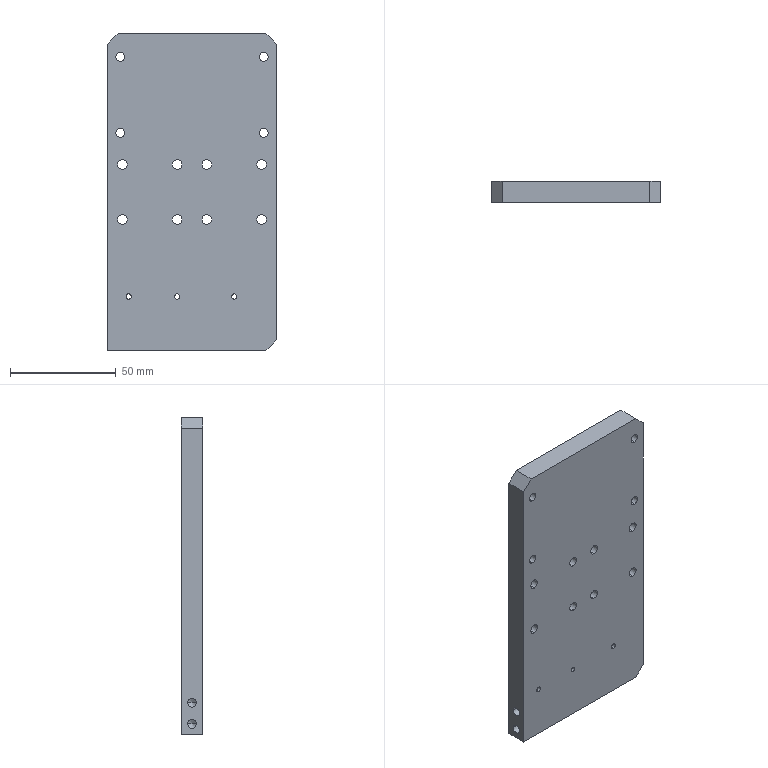Component | SolidWorks | F-YBExport-1-1_LSDH-6-025-1 | 1 solid | 79 faces | box 80 x 10 x 150 mm | volume 115928 mm3 | cylinder 54 | plane 17 | cone 8 | commonest cylinder face diameters 8 x16 4.5 x16 4.2 x12 2.5 x6 3 x4
build123d program:
from build123d import *

# Parameters (mm, degrees)
SKETCH1_W                                            = 150
SKETCH1_H                                            = 80
BOSS_EXTRUDE1_DEPTH                                  = 10
M3_TAPPED_HOLE1_D                                    = 2.5
HOLE_SIZE_ACCORDING_TO_THE_TYPE_OF_HEX_S_D           = 4.5
HOLE_SIZE_ACCORDING_TO_THE_TYPE_OF_HEX_S_CBORE_D     = 8
HOLE_SIZE_ACCORDING_TO_THE_TYPE_OF_HEX_S_CBORE_DEPTH = 4.6
M5_TAPPED_HOLE1_D                                    = 4.2
M5_TAPPED_HOLE1_DEPTH                                = 12.4
M5_TAPPED_HOLE1_TIP                                  = 1.262
M5_TAPPED_HOLE2_D                                    = 4.2
M5_TAPPED_HOLE2_DEPTH                                = 12.4
M5_TAPPED_HOLE2_TIP                                  = 1.262
F_3_0_3_DIAMETER_HOLE1_D                             = 3
F_3_0_3_DIAMETER_HOLE1_DEPTH                         = 7
F_3_0_3_DIAMETER_HOLE1_TIP                           = 0.9013
CHAMFER1_SIZE                                        = 5


with BuildPart() as part:
    # Sketch1 → Boss-Extrude1 (new body)
    with BuildSketch(Plane.XY):
        Rectangle(SKETCH1_W, SKETCH1_H)
    extrude(amount=BOSS_EXTRUDE1_DEPTH)

    # M3 Tapped Hole1 (through all)
    with Locations(Plane(origin=(49.5, 7, 10), x_dir=(1, 0, 0), z_dir=(0, 0, 1))):
        with Locations((0, 0), (0, -27), (0, 23)):
            Hole(M3_TAPPED_HOLE1_D / 2)

    # Hole size according to the type of hex s (through all)
    with Locations(Plane(origin=(-13, 33, 10), x_dir=(1, 0, 0), z_dir=(0, 0, 1))):
        with Locations((0, 0), (26, 0), (0, -26), (26, -26), (0, -40), (26, -40), (0, -66), (26, -66)):
            CounterBoreHole(HOLE_SIZE_ACCORDING_TO_THE_TYPE_OF_HEX_S_D / 2, HOLE_SIZE_ACCORDING_TO_THE_TYPE_OF_HEX_S_CBORE_D / 2, HOLE_SIZE_ACCORDING_TO_THE_TYPE_OF_HEX_S_CBORE_DEPTH)

    # M5 Tapped Hole1
    with Locations(Plane(origin=(60, 40, 5), x_dir=(0, 0, 1), z_dir=(0, 1, 0))):
        with Locations((0, 0), (0, 10)):
            Hole(M5_TAPPED_HOLE1_D / 2, depth=M5_TAPPED_HOLE1_DEPTH)
            with Locations((0, 0, -(M5_TAPPED_HOLE1_DEPTH + M5_TAPPED_HOLE1_TIP / 2))):  # 118° drill point
                Cone(0, M5_TAPPED_HOLE1_D / 2, M5_TAPPED_HOLE1_TIP, mode=Mode.SUBTRACT)

    # M5 Tapped Hole2
    with Locations(Plane(origin=(-64, 34, 10), x_dir=(1, 0, 0), z_dir=(0, 0, 1))):
        with Locations((0, 0), (36, 0), (0, -68), (36, -68)):
            Hole(M5_TAPPED_HOLE2_D / 2, depth=M5_TAPPED_HOLE2_DEPTH)
            with Locations((0, 0, -(M5_TAPPED_HOLE2_DEPTH + M5_TAPPED_HOLE2_TIP / 2))):  # 118° drill point
                Cone(0, M5_TAPPED_HOLE2_D / 2, M5_TAPPED_HOLE2_TIP, mode=Mode.SUBTRACT)

    # 3.0 _3_ Diameter Hole1
    with Locations(Plane(origin=(-61, 0, 10), x_dir=(1, 0, 0), z_dir=(0, 0, 1))):
        with Locations((0, 0), (30, 0)):
            Hole(F_3_0_3_DIAMETER_HOLE1_D / 2, depth=F_3_0_3_DIAMETER_HOLE1_DEPTH)
            with Locations((0, 0, -(F_3_0_3_DIAMETER_HOLE1_DEPTH + F_3_0_3_DIAMETER_HOLE1_TIP / 2))):  # 118° drill point
                Cone(0, F_3_0_3_DIAMETER_HOLE1_D / 2, F_3_0_3_DIAMETER_HOLE1_TIP, mode=Mode.SUBTRACT)

    # Chamfer1
    chamfer1_edges = [part.edges().sort_by_distance(p)[0] for p in [
        (75, -40, 5),
        (-75, -40, 5),
        (-75, 40, 5),
    ]]
    chamfer(chamfer1_edges, length=CHAMFER1_SIZE)


solid = part.part

# Placed as in the assembly
solid = solid.moved(Location((329.305, 320.175, 129.979), (-90, 0, 90)))